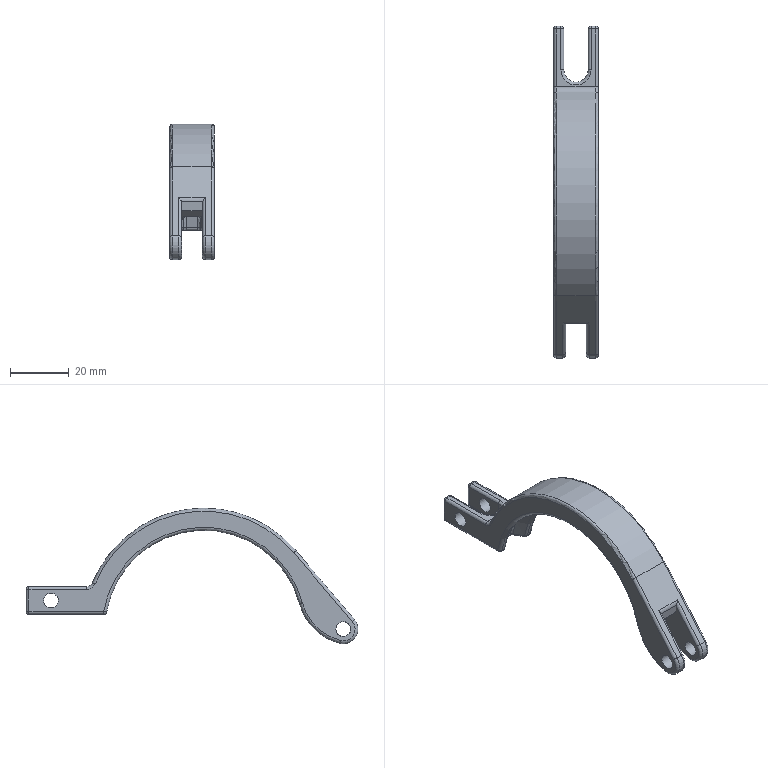Component | NX | TOP_BUCKLE | 1 solid | 100 faces | volume 11609 mm3 | cylinder 39 | torus 22 | sphere 14 | plane 13 | spline 10 | cone 2 | commonest cylinder face diameters 2 x24 5.1 x4 10 x2 38.209 x2 67.5 x2 4 x2 82.5 x1 8.3 x1